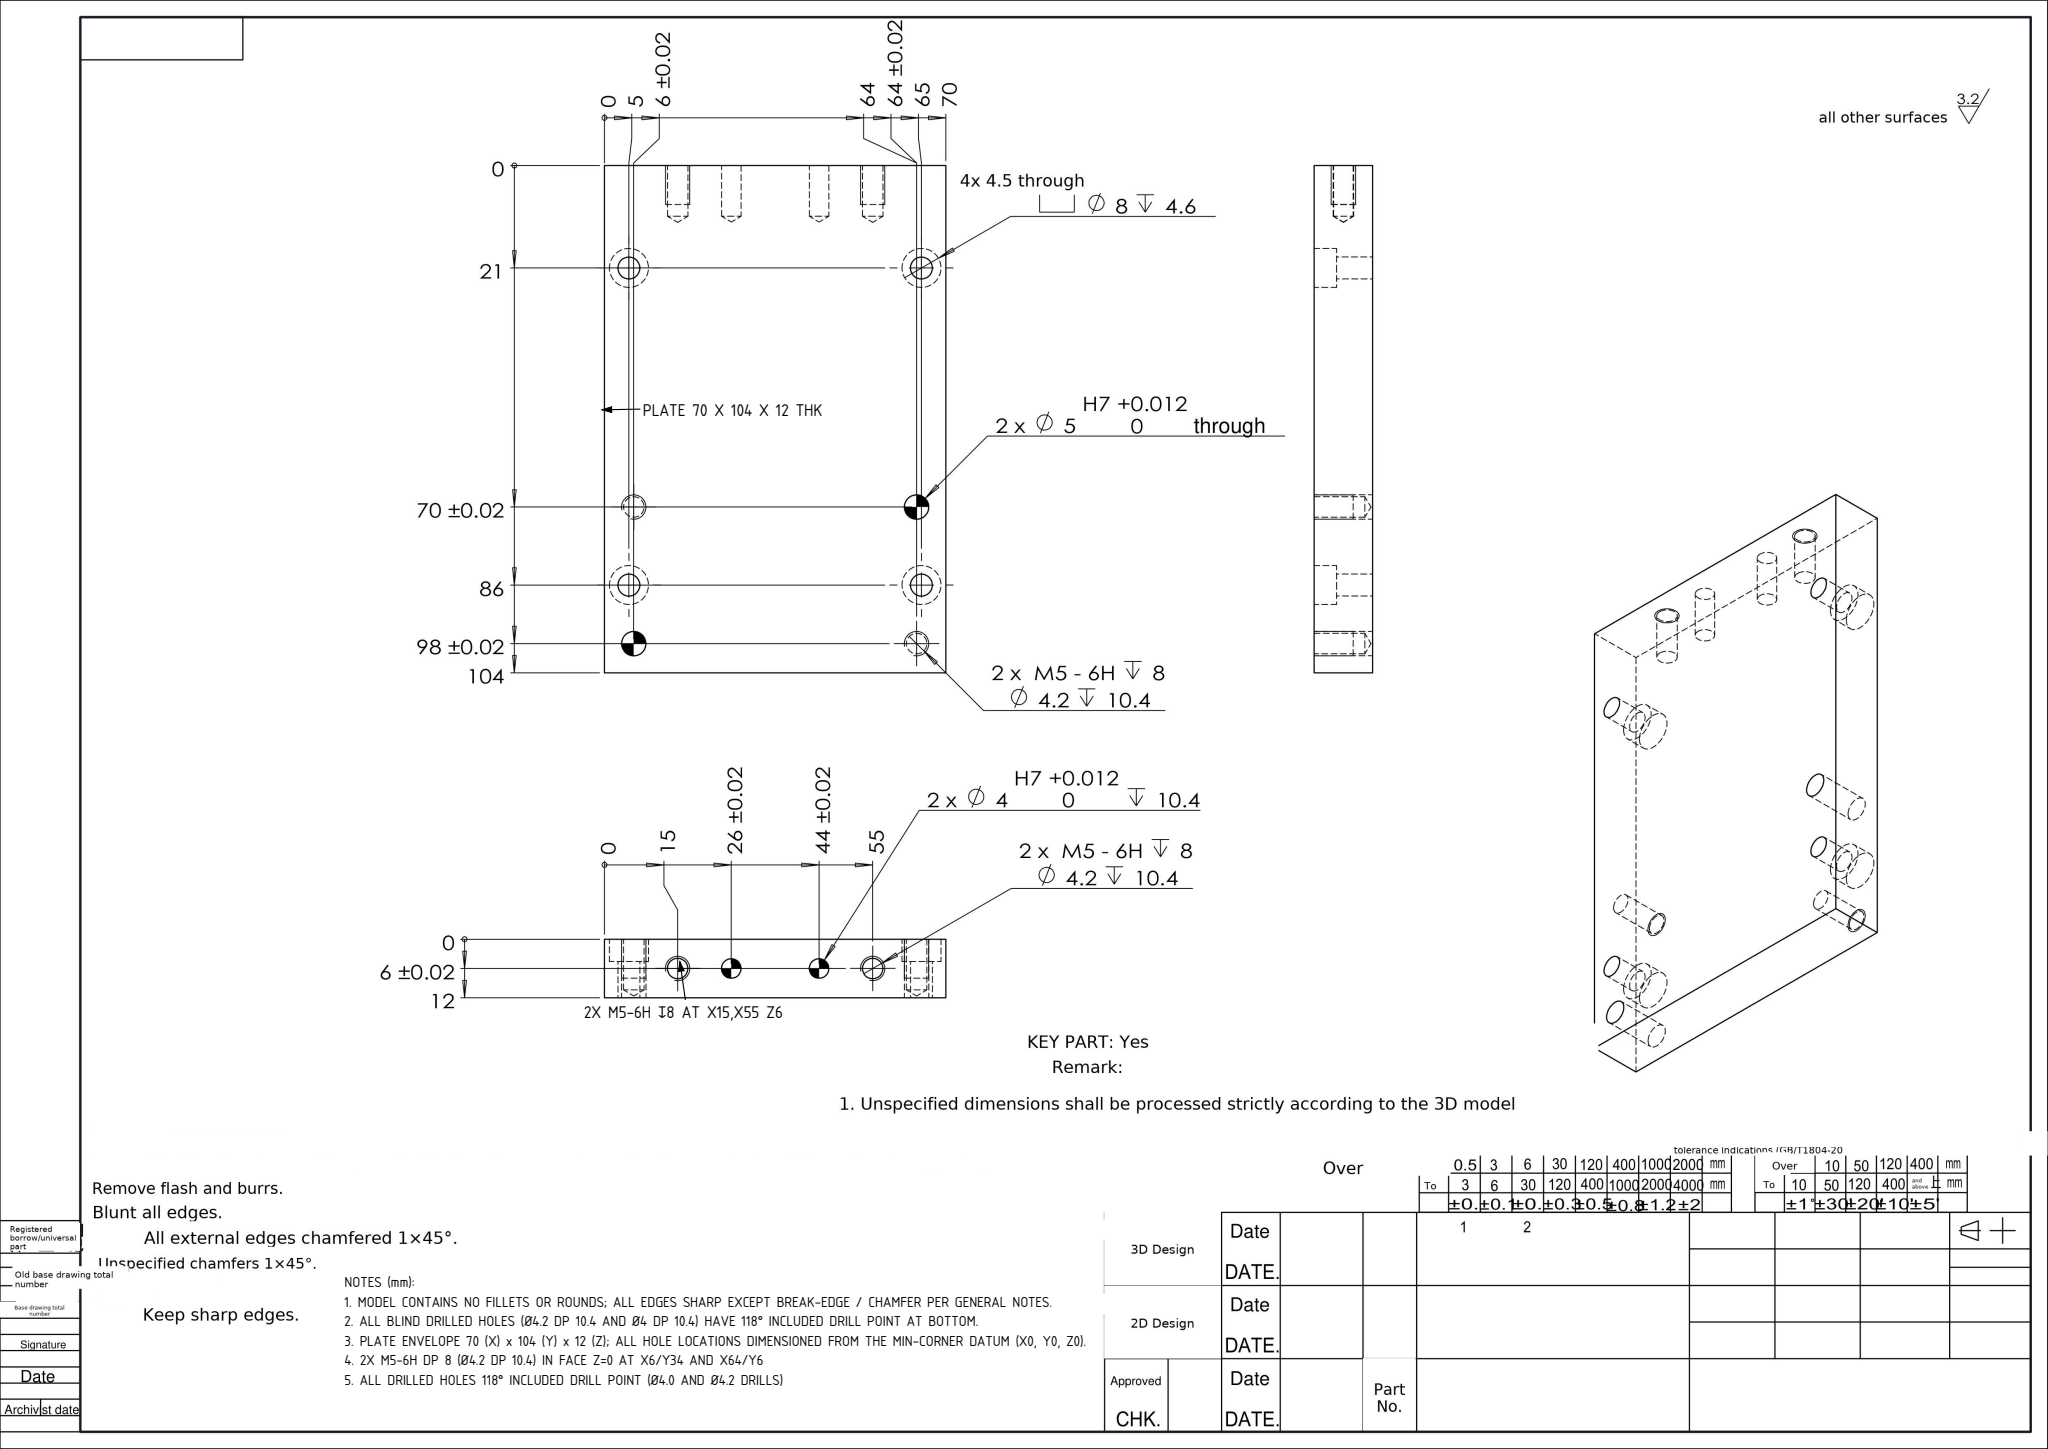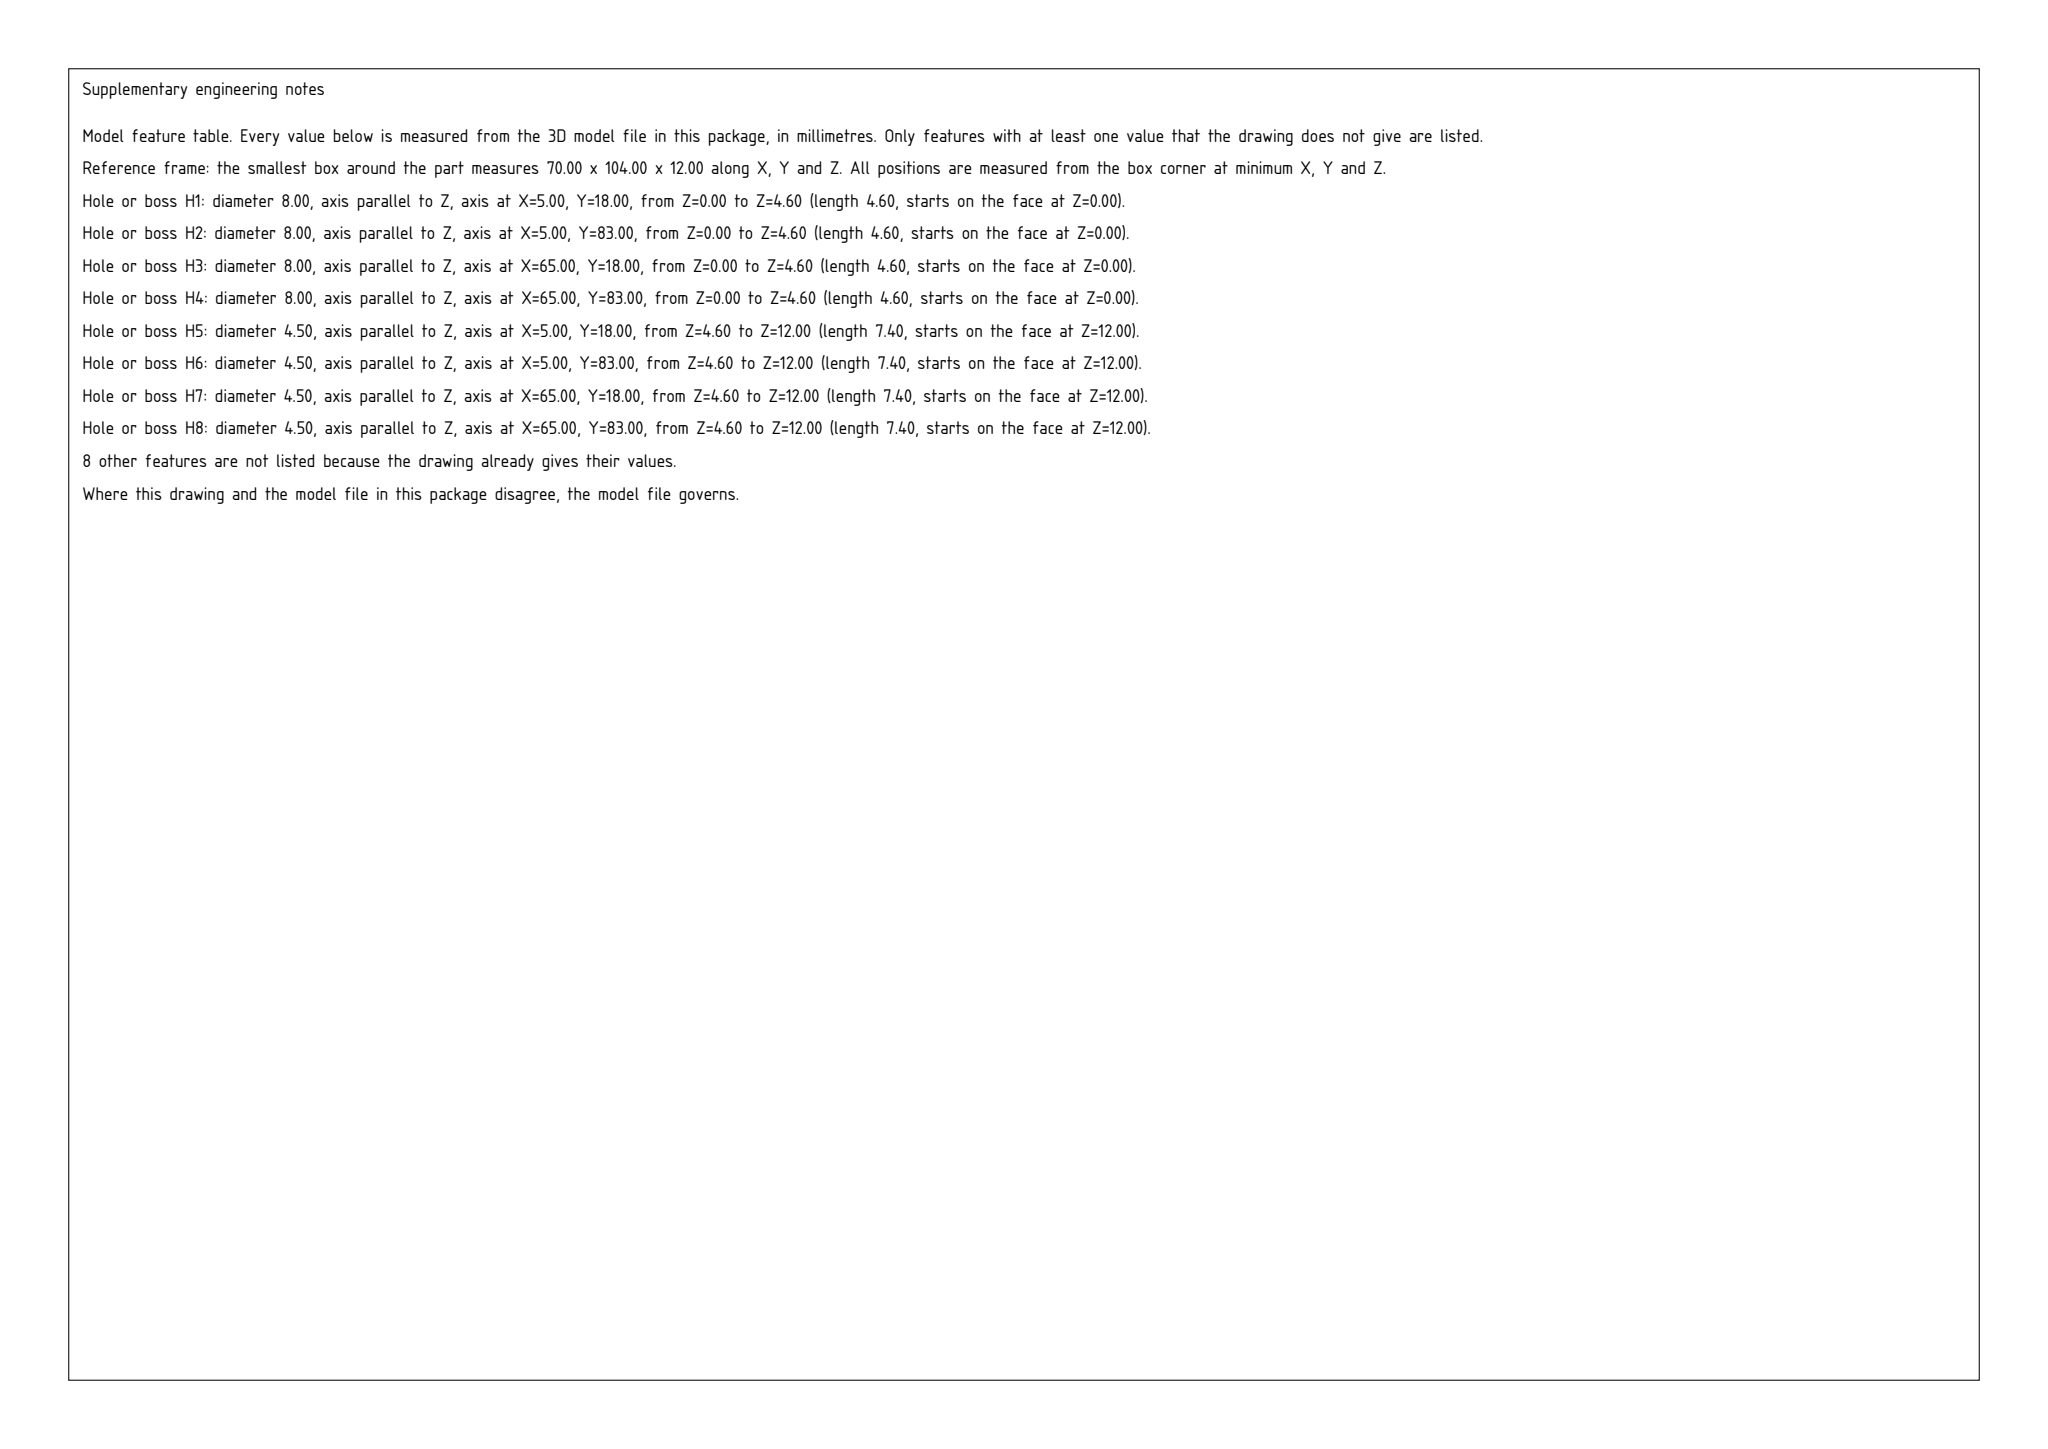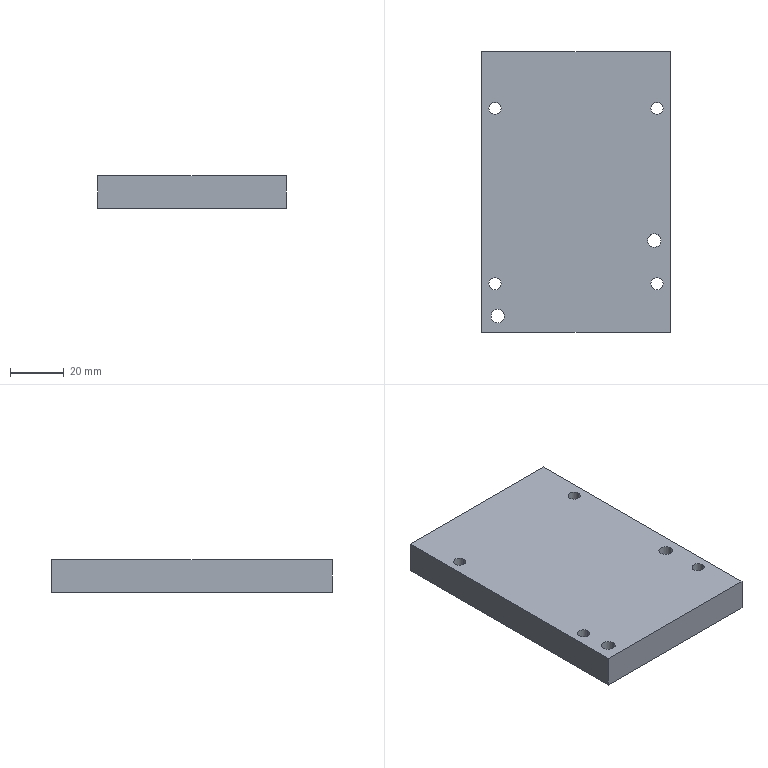Part | SolidWorks | mm | material 45 | 1 solid | 54 faces | box 70 x 104 x 12 mm | volume 84622 mm3 | cylinder 32 | cone 12 | plane 10 | commonest cylinder face diameters 4.2 x8 8 x8 4.5 x8 5 x4 4 x4
Drawing notes:
MODEL CONTAINS NO FILLETS OR ROUNDS; ALL EDGES SHARP EXCEPT BREAK-EDGE / CHAMFER PER GENERAL NOTES. | from the solid: fillet_radii: [] (empty list)
ALL BLIND DRILLED HOLES (Ø4.2 DP 10.4 AND Ø4 DP 10.4) HAVE 118° INCLUDED DRILL POINT AT BOTTOM. | from the solid: cones[included_angle,ref_dia]: [118.0, 4.2, 8] and [118.0, 4.0, 4]
PLATE ENVELOPE 70 (X) x 104 (Y) x 12 (Z); ALL HOLE LOCATIONS DIMENSIONED FROM THE MIN-CORNER DATUM (X0, Y0, Z0). | from the solid: bbox_xyz [70.0, 104.0, 12.0]; axis_planes x 0/70, y 0/104, z 0/12
PLATE OVERALL 70 WIDE x 104 LONG x 12 THK; ALL HOLE LOCATIONS FROM BOTTOM-LEFT CORNER (X0,Y0) OF THIS OUTLINE | from the solid: bbox_xyz [70.0,104.0,12.0] and origin_note 'positions are from min corner of bbox'
2X M5-6H DP 8 (Ø4.2 DP 10.4) IN FACE Z=0 AT X6/Y34 AND X64/Y6 | from the solid: cylinders [4.2,'z',[6.0,34.0,null],10.4] and [4.2,'z',[64.0,6.0,null],10.4]
2X M5-6H DP 8 (Ø4.2 DP 10.4) IN FACE Y=0 AT X15/Z6 AND X55/Z6 | from the solid: cylinders [4.2,'y',[15.0,null,6.0],10.4] and [4.2,'y',[55.0,null,6.0],10.4]
ALL DRILLED HOLES 118° INCLUDED DRILL POINT (Ø4.0 AND Ø4.2 DRILLS) | from the solid: cones [118.0,4.2] and [118.0,4.0]
build123d program:
from build123d import *

# Parameters (mm, degrees)
SKETCH1_W                                         = 70
SKETCH1_H                                         = 104
BOSS_EXTRUDE1_DEPTH                               = 12
HOLE_SIZE_ACCORDING_TO_HEXAGON_SOCKET_D           = 4.5
HOLE_SIZE_ACCORDING_TO_HEXAGON_SOCKET_CBORE_D     = 8
HOLE_SIZE_ACCORDING_TO_HEXAGON_SOCKET_CBORE_DEPTH = 4.6
M5_TAPPED_HOLE1_D                                 = 4.2
M5_TAPPED_HOLE1_DEPTH                             = 10.4
M5_TAPPED_HOLE1_TIP                               = 1.262
SIZE_MM_DOWEL_PIN_HOLE2_D                         = 4
SIZE_MM_DOWEL_PIN_HOLE2_DEPTH                     = 10.4
SIZE_MM_DOWEL_PIN_HOLE2_TIP                       = 1.202
M5_TAPPED_HOLE2_D                                 = 4.2
M5_TAPPED_HOLE2_DEPTH                             = 10.4
M5_TAPPED_HOLE2_TIP                               = 1.262
SIZE_MM_DOWEL_PIN_HOLE3_D                         = 5


with BuildPart() as part:
    # Sketch1 → Boss-Extrude1 (new body)
    with BuildSketch(Plane.XY):
        Rectangle(SKETCH1_W, SKETCH1_H)
    extrude(amount=BOSS_EXTRUDE1_DEPTH)

    # Hole Size _ according to_ Hexagon Socket (through all)
    with Locations(Plane(origin=(0, 0, 0), x_dir=(-1, 0, 0), z_dir=(0, 0, -1))):
        with Locations((30, -34), (30, 31), (-30, 31), (-30, -34)):
            CounterBoreHole(HOLE_SIZE_ACCORDING_TO_HEXAGON_SOCKET_D / 2, HOLE_SIZE_ACCORDING_TO_HEXAGON_SOCKET_CBORE_D / 2, HOLE_SIZE_ACCORDING_TO_HEXAGON_SOCKET_CBORE_DEPTH)

    # M5 Tapped Hole1
    with Locations(Plane(origin=(0, 52, 0), x_dir=(1, 0, 0), z_dir=(0, 1, 0))):
        with Locations((20, -6), (-20, -6)):
            Hole(M5_TAPPED_HOLE1_D / 2, depth=M5_TAPPED_HOLE1_DEPTH)
            with Locations((0, 0, -(M5_TAPPED_HOLE1_DEPTH + M5_TAPPED_HOLE1_TIP / 2))):  # 118° drill point
                Cone(0, M5_TAPPED_HOLE1_D / 2, M5_TAPPED_HOLE1_TIP, mode=Mode.SUBTRACT)

    # Size mm Dowel Pin Hole2
    with Locations(Plane(origin=(0, 52, 0), x_dir=(1, 0, 0), z_dir=(0, 1, 0))):
        with Locations((9, -6), (-9, -6)):
            Hole(SIZE_MM_DOWEL_PIN_HOLE2_D / 2, depth=SIZE_MM_DOWEL_PIN_HOLE2_DEPTH)
            with Locations((0, 0, -(SIZE_MM_DOWEL_PIN_HOLE2_DEPTH + SIZE_MM_DOWEL_PIN_HOLE2_TIP / 2))):  # 118° drill point
                Cone(0, SIZE_MM_DOWEL_PIN_HOLE2_D / 2, SIZE_MM_DOWEL_PIN_HOLE2_TIP, mode=Mode.SUBTRACT)

    # M5 Tapped Hole2
    with Locations(Plane(origin=(0, 0, 0), x_dir=(-1, 0, 0), z_dir=(0, 0, -1))):
        with Locations((-29, -46), (29, -18)):
            Hole(M5_TAPPED_HOLE2_D / 2, depth=M5_TAPPED_HOLE2_DEPTH)
            with Locations((0, 0, -(M5_TAPPED_HOLE2_DEPTH + M5_TAPPED_HOLE2_TIP / 2))):  # 118° drill point
                Cone(0, M5_TAPPED_HOLE2_D / 2, M5_TAPPED_HOLE2_TIP, mode=Mode.SUBTRACT)

    # Size mm Dowel Pin Hole3 (through all)
    with Locations(Plane(origin=(0, 0, 0), x_dir=(-1, 0, 0), z_dir=(0, 0, -1))):
        with Locations((-29, -18), (29, -46)):
            Hole(SIZE_MM_DOWEL_PIN_HOLE3_D / 2)


solid = part.part